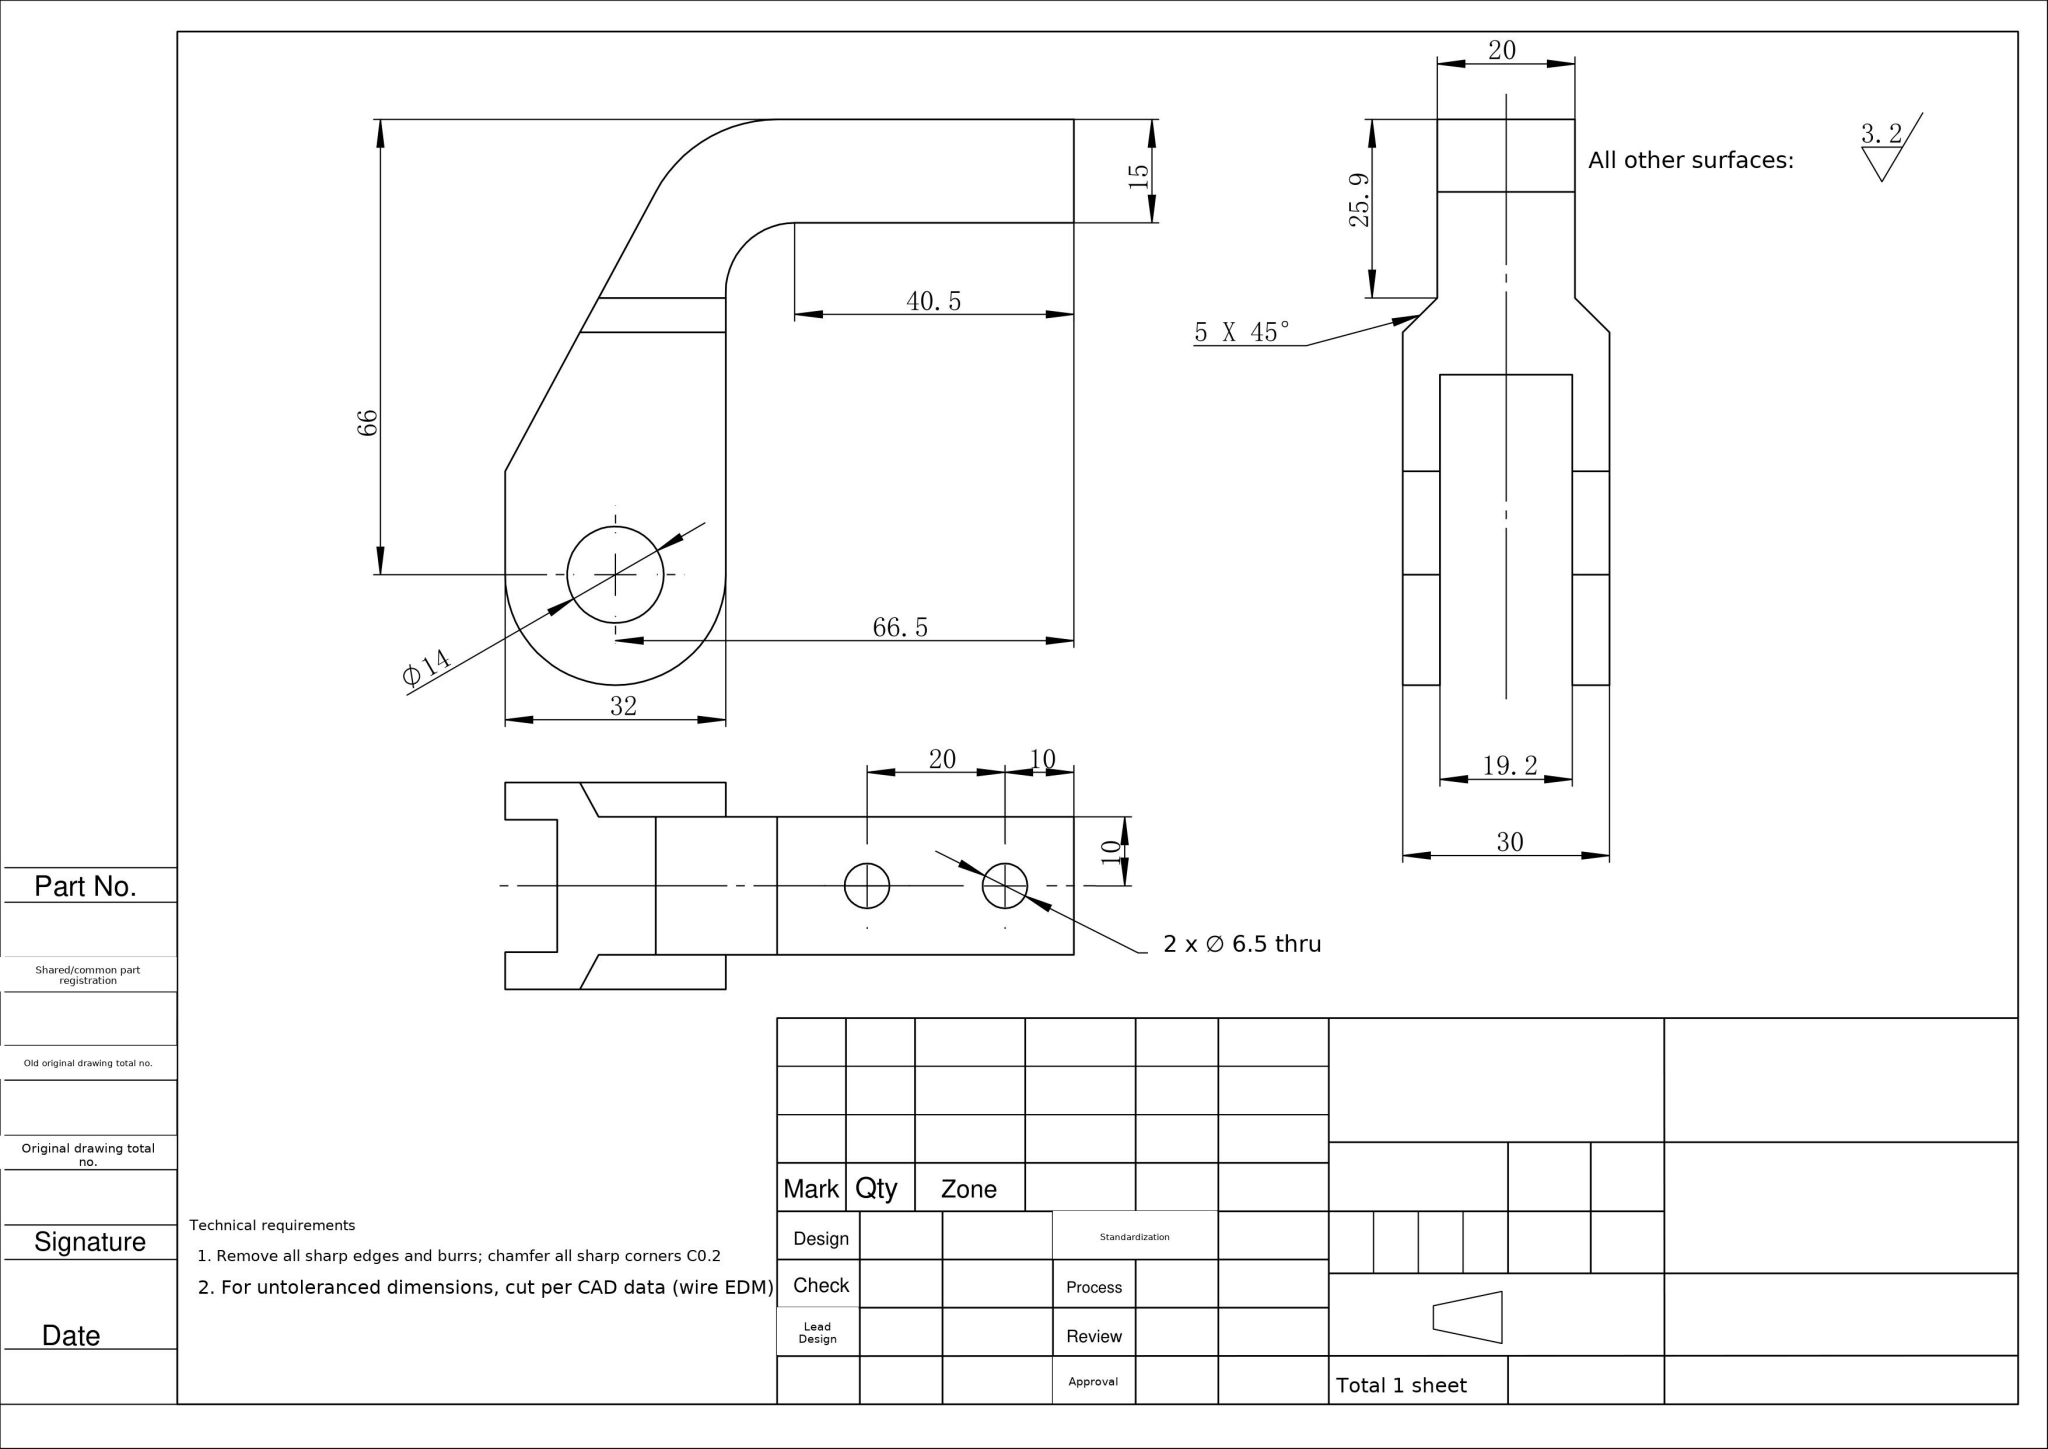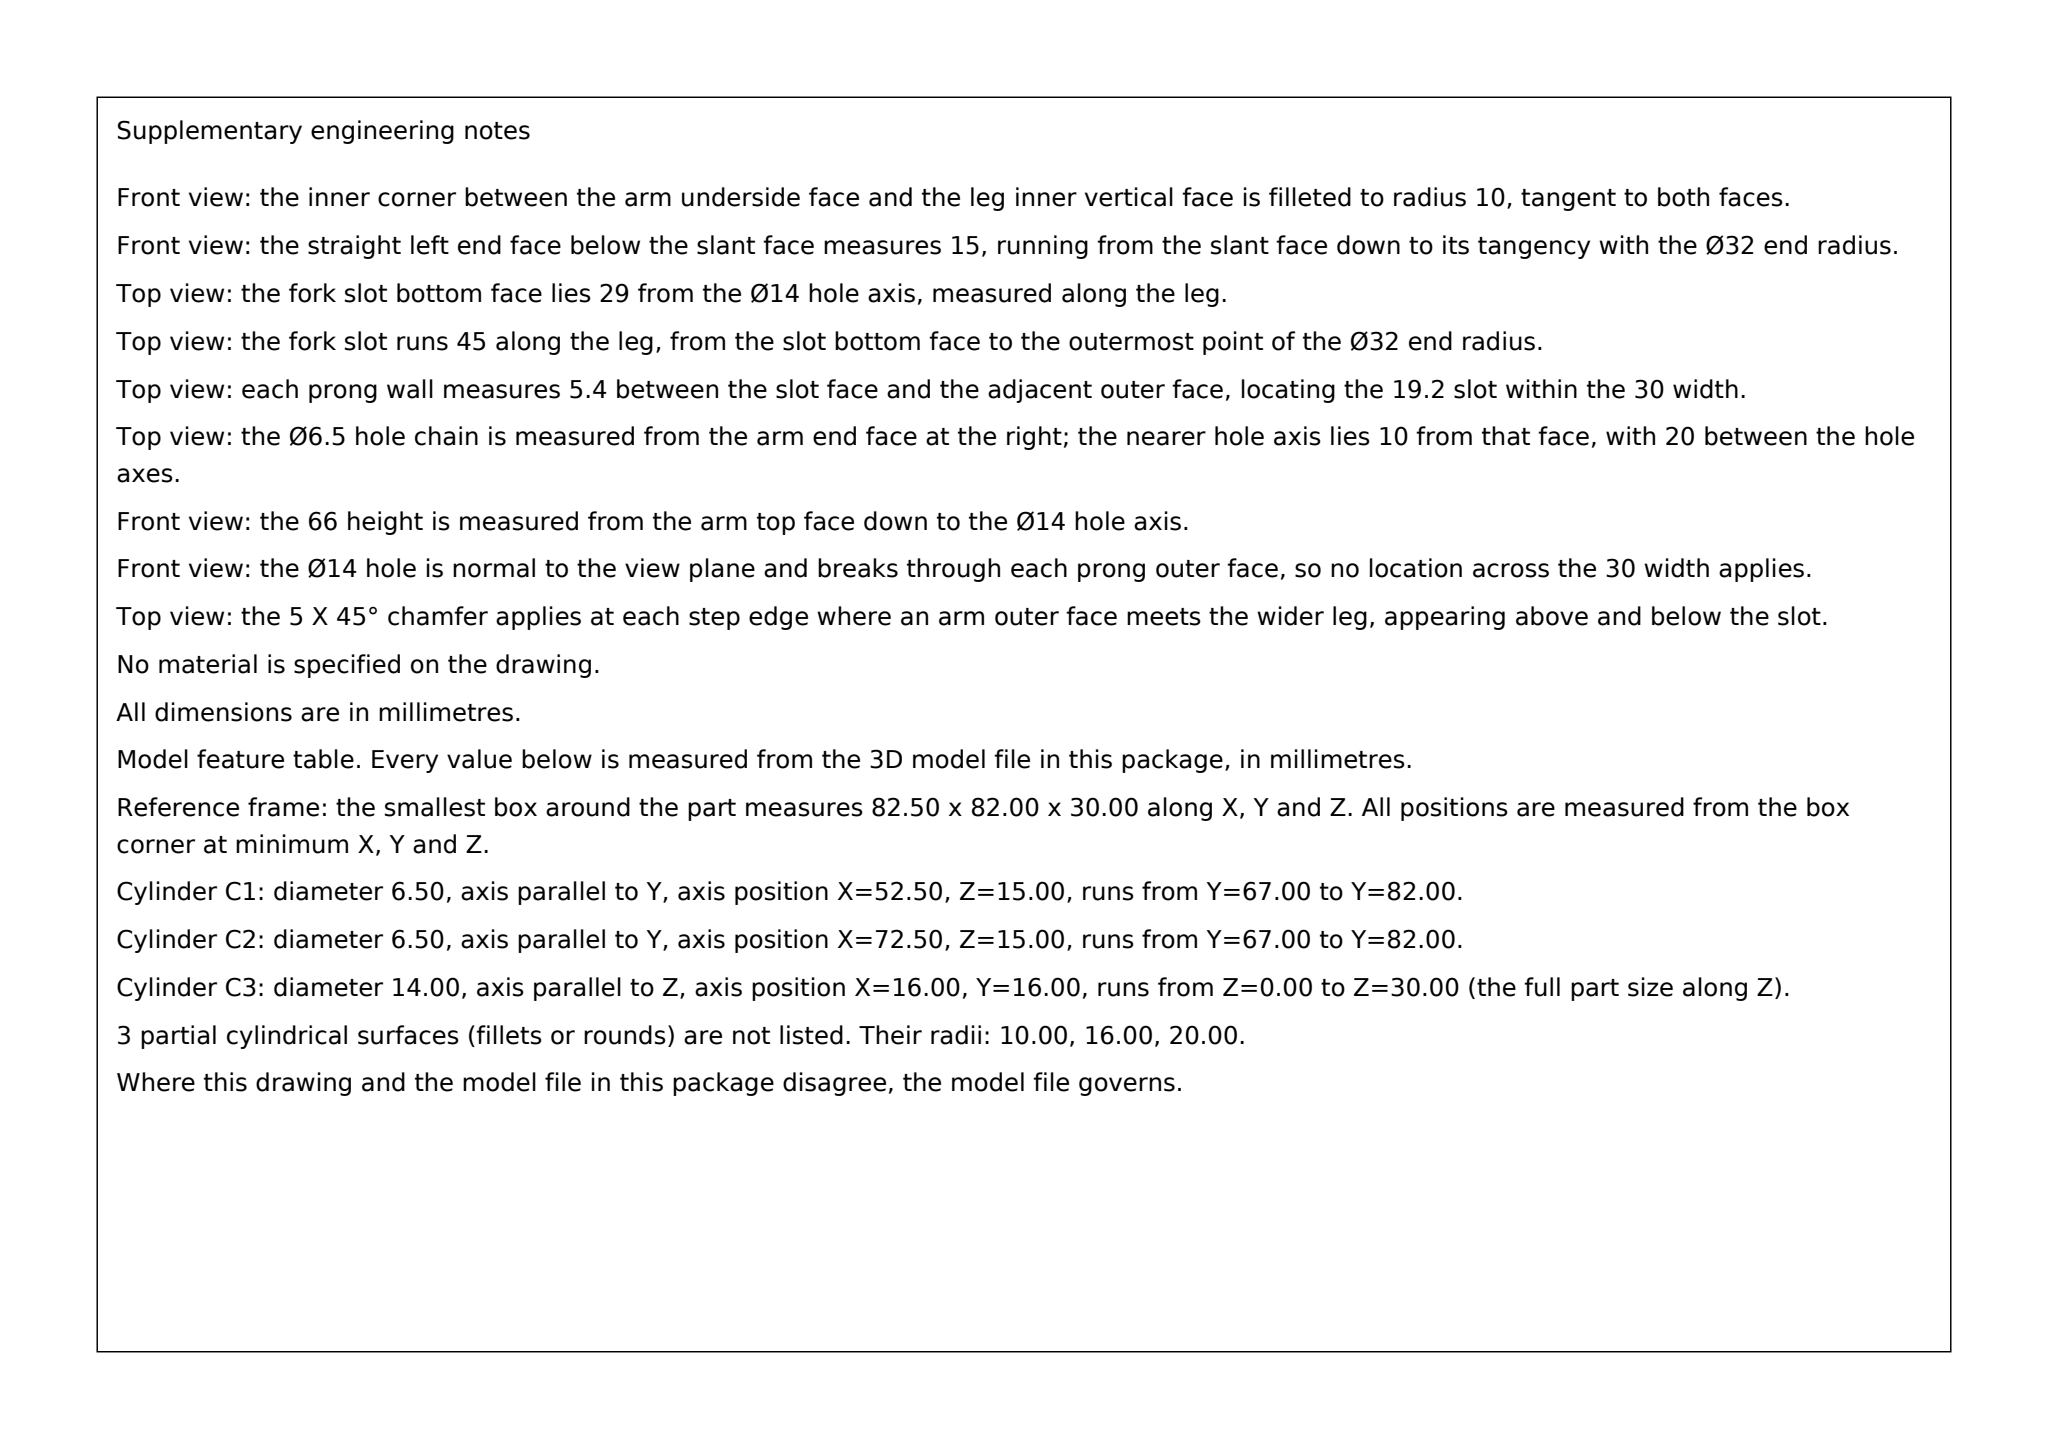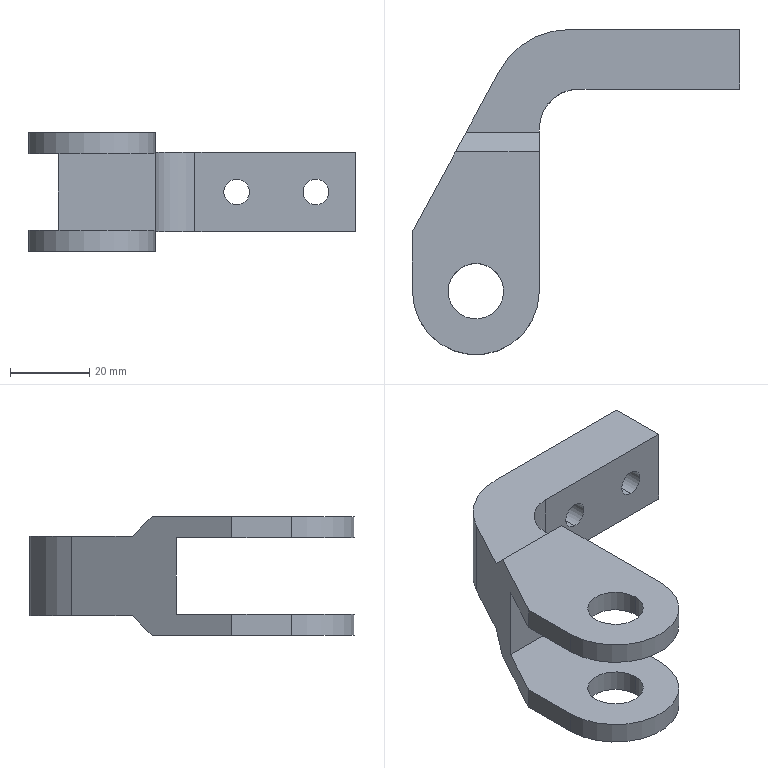Part | SolidWorks | mm | 1 solid | 28 faces | box 82.5 x 82 x 30 mm | volume 38860 mm3 | plane 16 | cylinder 12 | commonest cylinder face diameters 6.5 x4 14 x4 32 x2 20 x1 40 x1
Drawing notes:
FORK SLOT 19.2 WIDE x 45 DEEP FROM OPEN END | from the solid: axis_plane y=45 is slot end face; slot opens at y=0; width 19.2 dim on side view
R20 OUTER ARC: CTR 23.44 RT & 46 UP FROM Ø14 CL, TAN TOP FACE | from the solid: cyl dia 40 axis z at (39.44,62); O14 ctr (16,16); top face y=82 => 82-62=20=R
R10 INNER ARC: CTR 40.5 FROM RH EDGE, TAN TO 15 ARM UNDERSIDE | from the solid: cyl dia 20 axis z at (42,57); bbox x=82.5 => 40.5; plane y=67 => 67-57=10=R
SLANT EDGE 67.44 DEG TO HORIZ, TAN TO R16 TAB & R20 ARC | from the solid: common ext tangent of dia32 at (16,16) and dia40 at (39.44,62): 67.44 deg